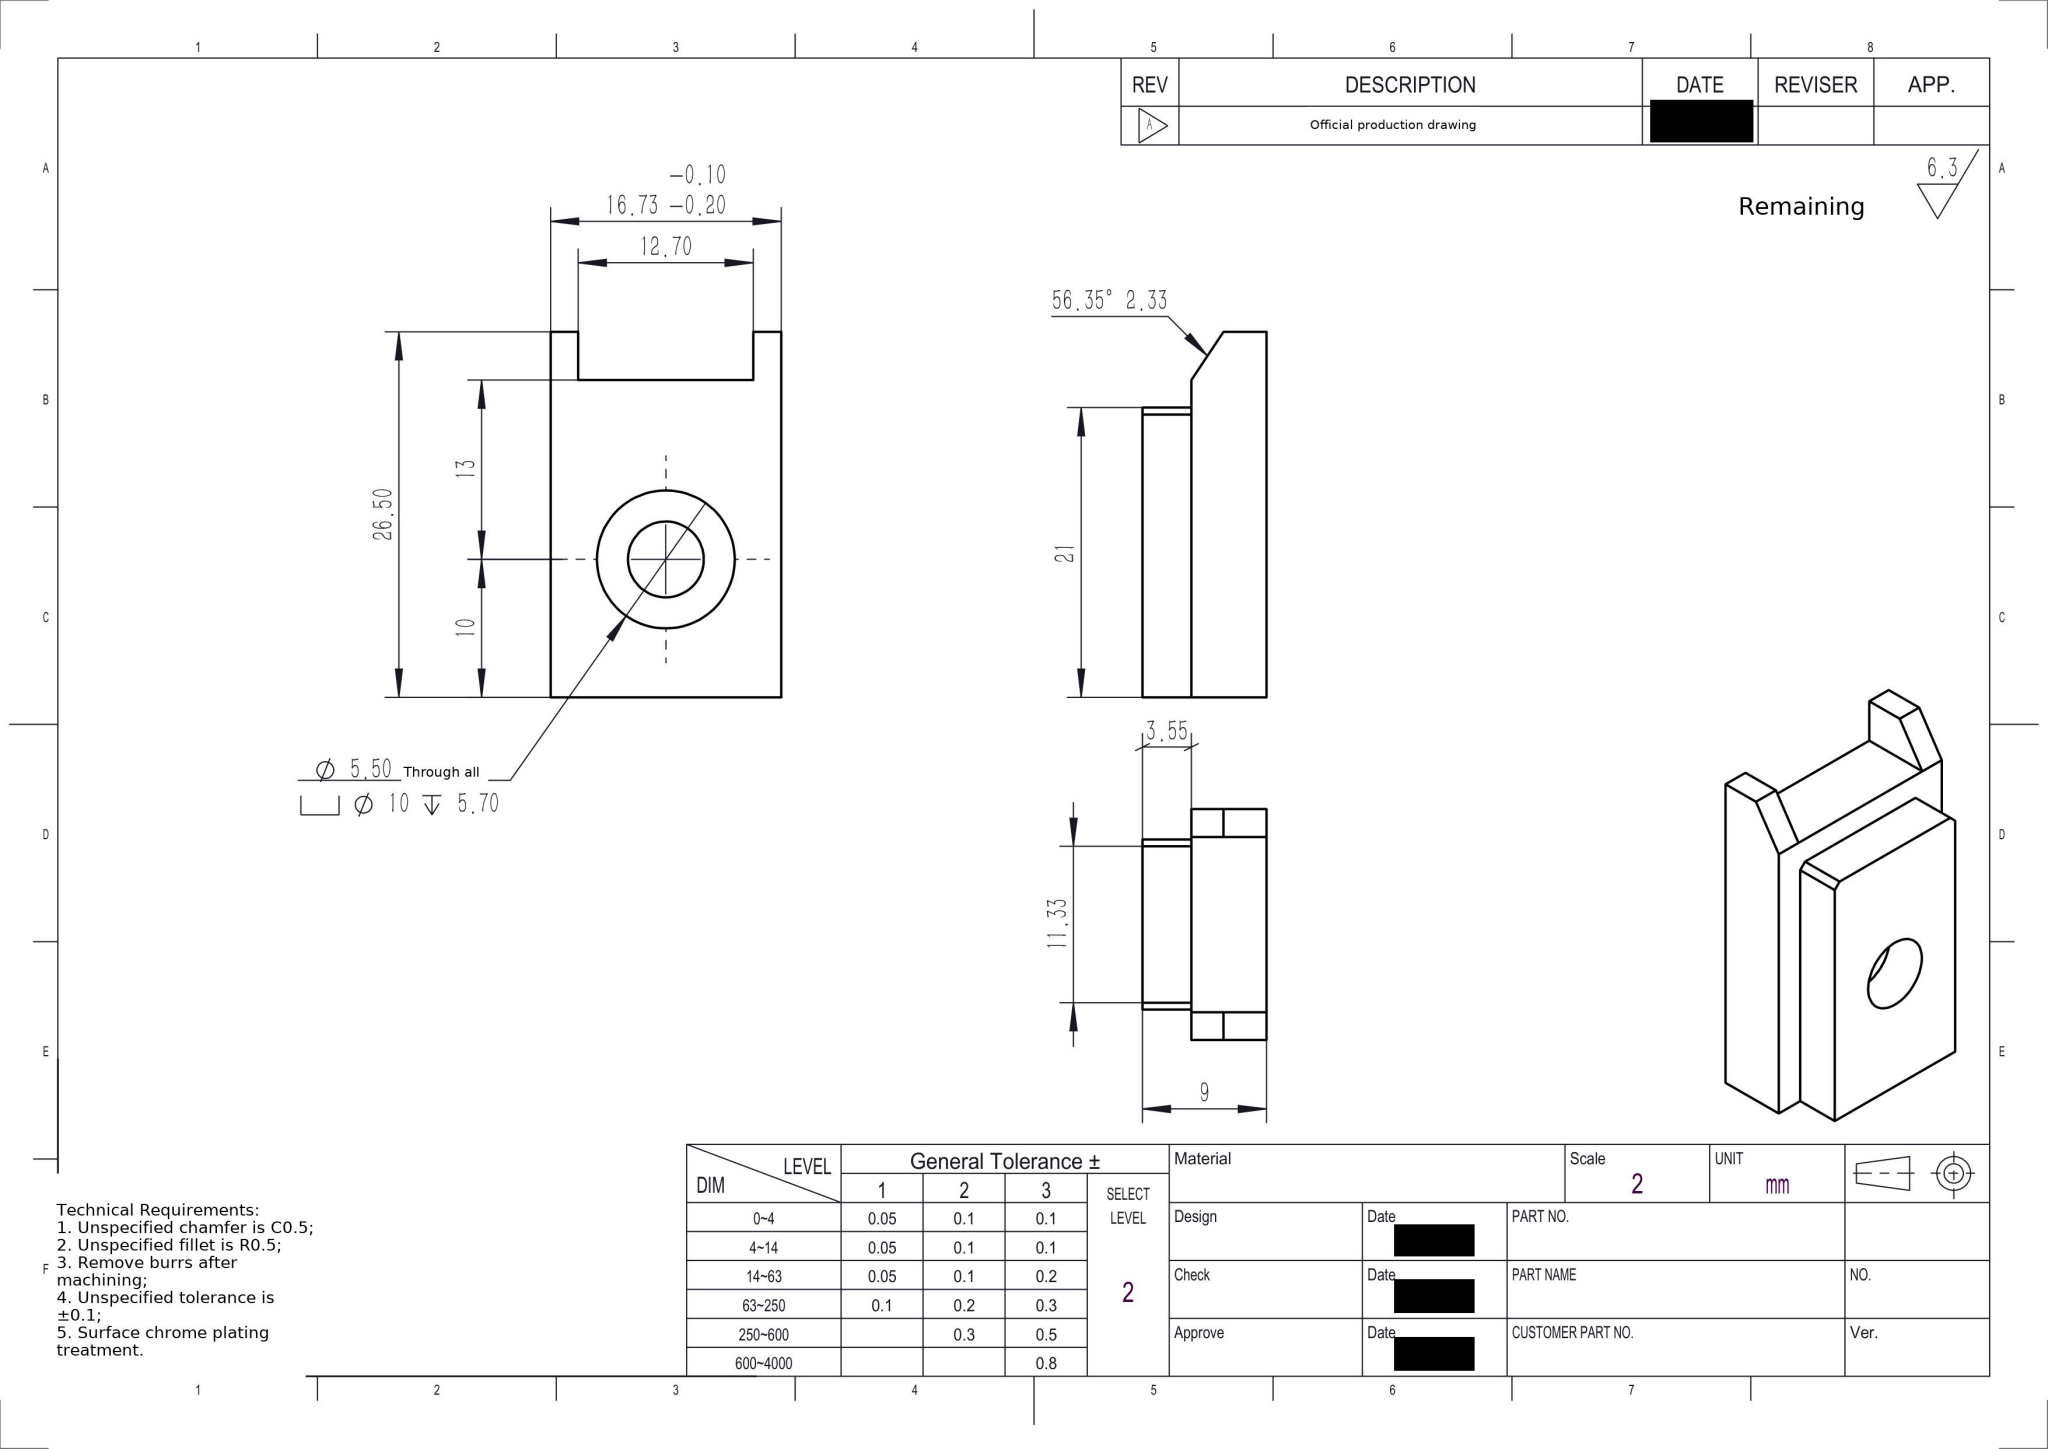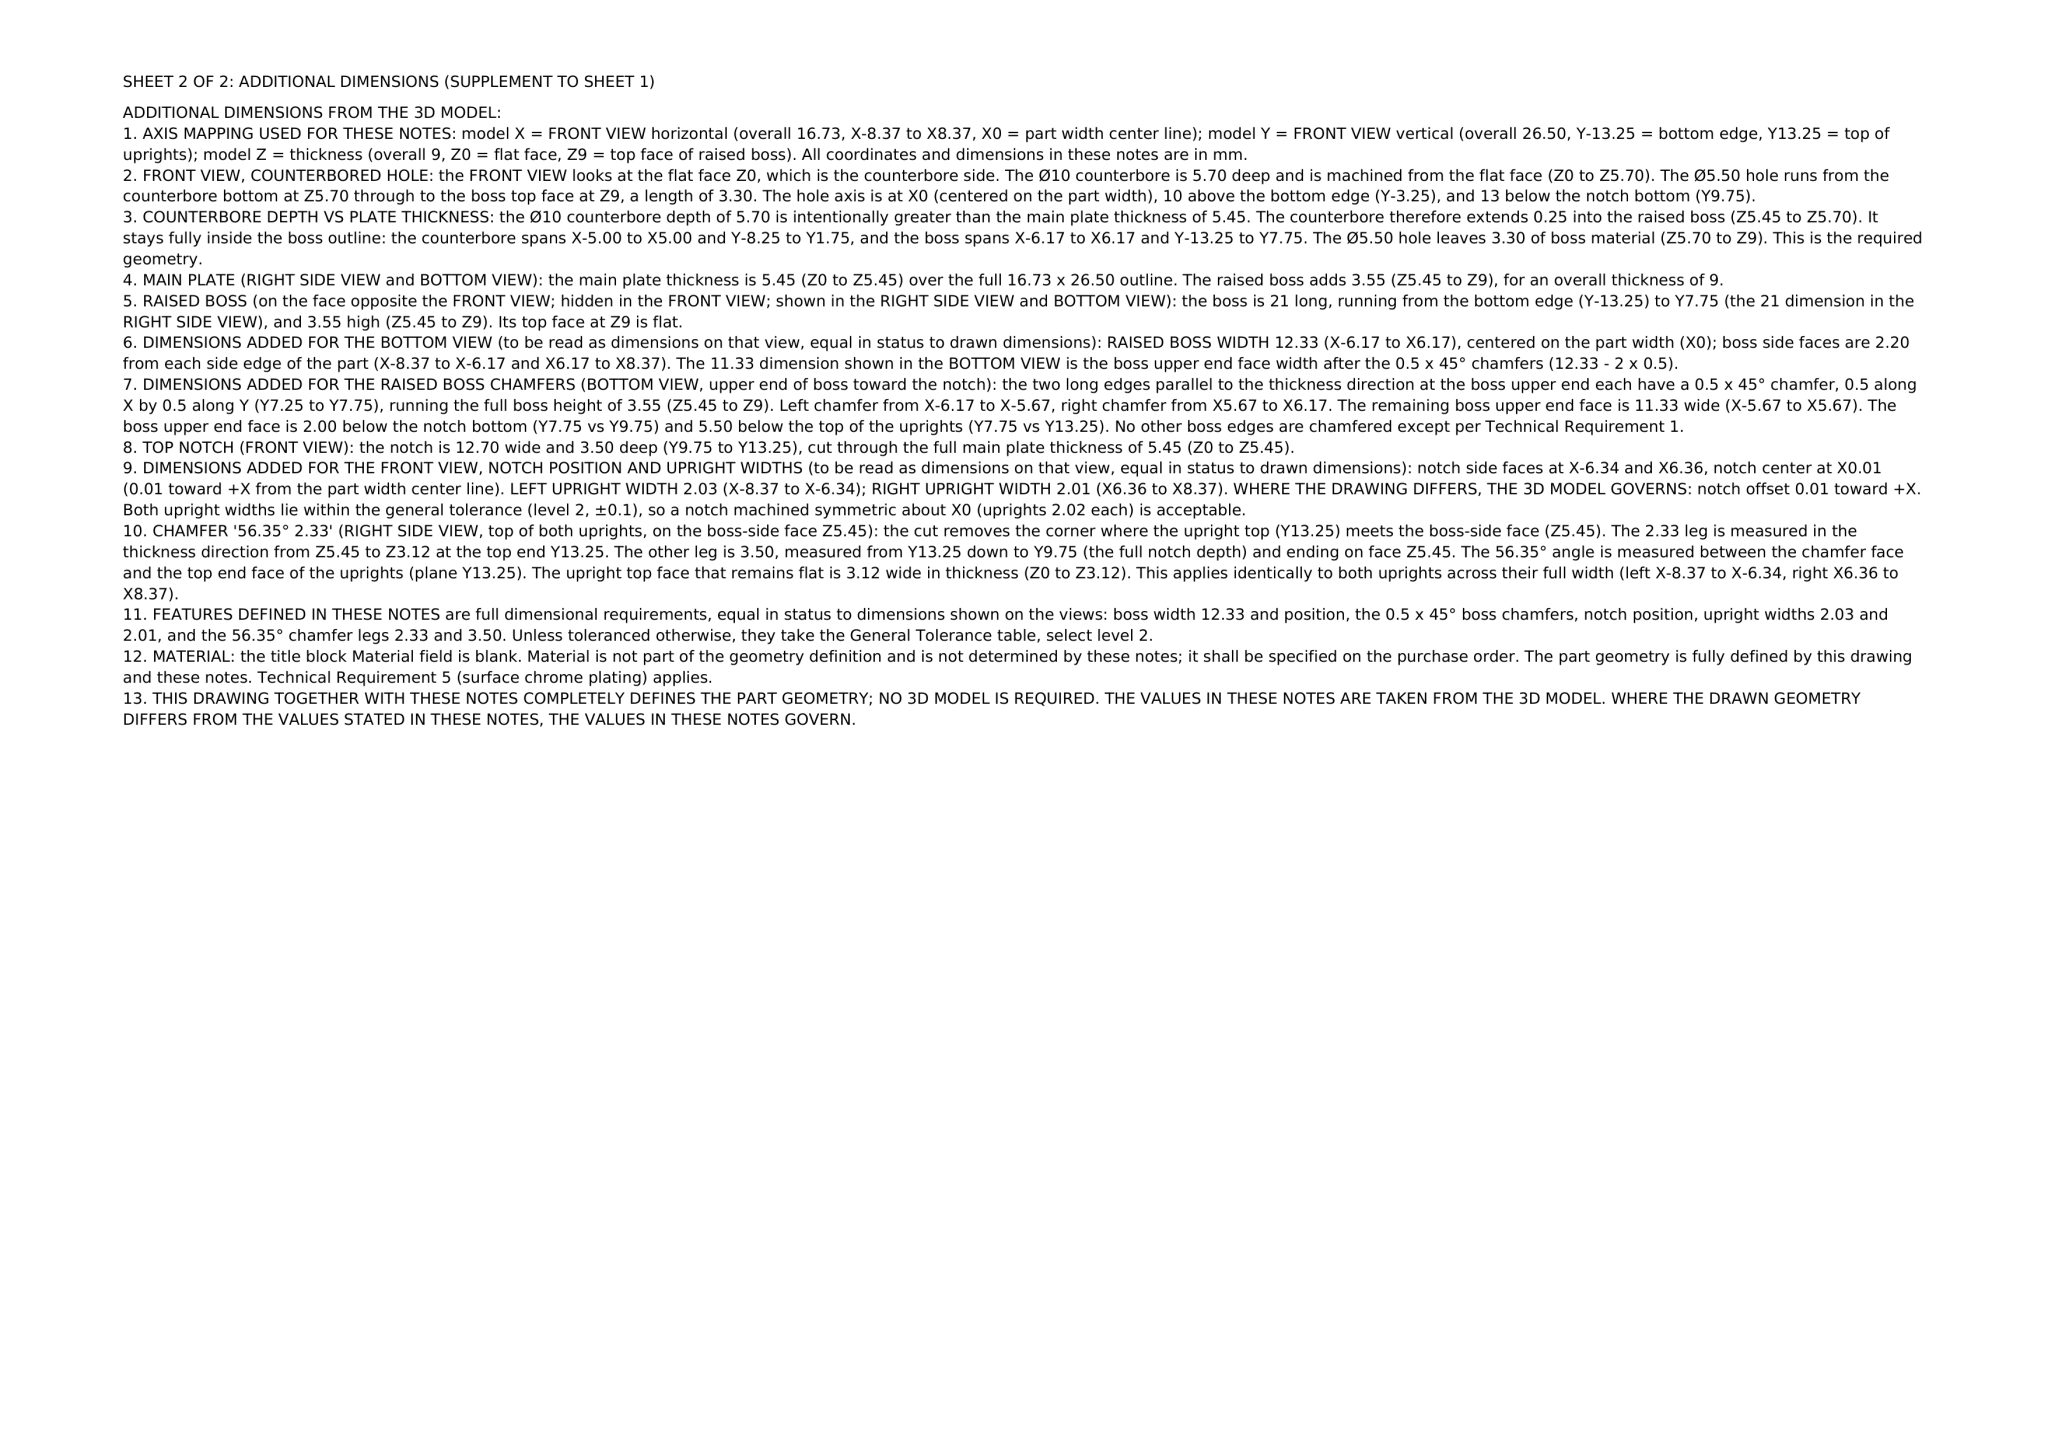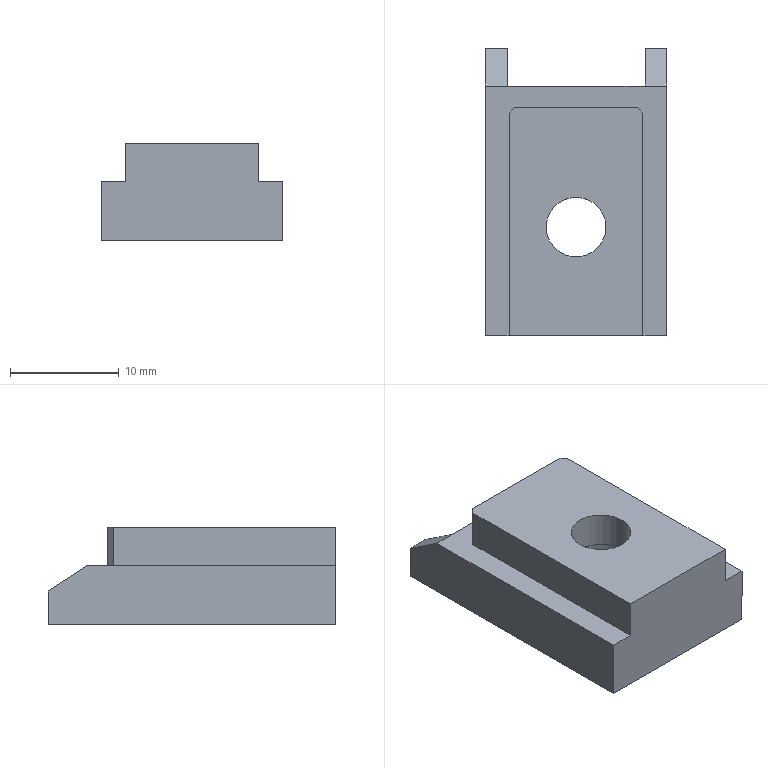Part | NX | mm | 396 | 1 solid | 23 faces | box 16.73 x 26.5 x 9 mm | volume 2550 mm3 | plane 19 | cylinder 4 | commonest cylinder face diameters 10 x2 5.5 x2
STEP:
#1=COLOUR_RGB('',0.7765,0.7569,0.7373);
#2=FILL_AREA_STYLE_COLOUR('',#1);
#3=FILL_AREA_STYLE('',(#2));
#4=SURFACE_STYLE_FILL_AREA(#3);
#5=SURFACE_SIDE_STYLE('',(#4));
#6=SURFACE_STYLE_USAGE(.BOTH.,#5);
#7=PRESENTATION_STYLE_ASSIGNMENT((#6));
#8=CARTESIAN_POINT('',(5.005,-3.25,5.7));
#9=VERTEX_POINT('',#8);
#10=CARTESIAN_POINT('',(-4.995,-3.25,5.7));
#11=VERTEX_POINT('',#10);
#12=CARTESIAN_POINT('',(0.005,-3.25,5.7));
#13=DIRECTION('',(0.,0.,-1.));
#14=DIRECTION('',(-1.,0.,0.));
#15=AXIS2_PLACEMENT_3D('',#12,#13,#14);
#16=CIRCLE('',#15,5.);
#17=EDGE_CURVE('',#9,#11,#16,.T.);
#18=ORIENTED_EDGE('',*,*,#17,.F.);
#19=CARTESIAN_POINT('',(5.005,-3.25,-0.));
#20=VERTEX_POINT('',#19);
#21=CARTESIAN_POINT('',(5.005,-3.25,0.));
#22=DIRECTION('',(0.,0.,-1.));
#23=VECTOR('',#22,1000.);
#24=LINE('',#21,#23);
#25=EDGE_CURVE('',#9,#20,#24,.T.);
#26=ORIENTED_EDGE('',*,*,#25,.T.);
#27=CARTESIAN_POINT('',(-4.995,-3.25,-0.));
#28=VERTEX_POINT('',#27);
#29=CARTESIAN_POINT('',(0.005,-3.25,-0.));
#30=DIRECTION('',(0.,0.,-1.));
#31=DIRECTION('',(-1.,0.,0.));
#32=AXIS2_PLACEMENT_3D('',#29,#30,#31);
#33=CIRCLE('',#32,5.);
#34=EDGE_CURVE('',#20,#28,#33,.T.);
#35=ORIENTED_EDGE('',*,*,#34,.T.);
#36=CARTESIAN_POINT('',(-4.995,-3.25,0.));
#37=DIRECTION('',(0.,0.,-1.));
#38=VECTOR('',#37,1000.);
#39=LINE('',#36,#38);
#40=EDGE_CURVE('',#11,#28,#39,.T.);
#41=ORIENTED_EDGE('',*,*,#40,.F.);
#42=EDGE_LOOP('',(#18,#26,#35,#41));
#43=FACE_OUTER_BOUND('',#42,.T.);
#44=CARTESIAN_POINT('',(0.005,-3.25,0.));
#45=DIRECTION('',(0.,0.,-1.));
#46=DIRECTION('',(-1.,0.,0.));
#47=AXIS2_PLACEMENT_3D('',#44,#45,#46);
#48=CYLINDRICAL_SURFACE('',#47,5.);
#49=ADVANCED_FACE('',(#43),#48,.F.);
#50=CARTESIAN_POINT('',(2.755,-3.25,9.));
#51=VERTEX_POINT('',#50);
#52=CARTESIAN_POINT('',(-2.745,-3.25,9.));
#53=VERTEX_POINT('',#52);
#54=CARTESIAN_POINT('',(0.005,-3.25,9.));
#55=DIRECTION('',(0.,0.,-1.));
#56=DIRECTION('',(-1.,0.,0.));
#57=AXIS2_PLACEMENT_3D('',#54,#55,#56);
#58=CIRCLE('',#57,2.75);
#59=EDGE_CURVE('',#51,#53,#58,.T.);
#60=ORIENTED_EDGE('',*,*,#59,.F.);
#61=CARTESIAN_POINT('',(2.755,-3.25,5.7));
#62=VERTEX_POINT('',#61);
#63=CARTESIAN_POINT('',(2.755,-3.25,0.));
#64=DIRECTION('',(0.,0.,-1.));
#65=VECTOR('',#64,1000.);
#66=LINE('',#63,#65);
#67=EDGE_CURVE('',#51,#62,#66,.T.);
#68=ORIENTED_EDGE('',*,*,#67,.T.);
#69=CARTESIAN_POINT('',(-2.745,-3.25,5.7));
#70=VERTEX_POINT('',#69);
#71=CARTESIAN_POINT('',(0.005,-3.25,5.7));
#72=DIRECTION('',(0.,0.,-1.));
#73=DIRECTION('',(-1.,0.,0.));
#74=AXIS2_PLACEMENT_3D('',#71,#72,#73);
#75=CIRCLE('',#74,2.75);
#76=EDGE_CURVE('',#62,#70,#75,.T.);
#77=ORIENTED_EDGE('',*,*,#76,.T.);
#78=CARTESIAN_POINT('',(-2.745,-3.25,0.));
#79=DIRECTION('',(0.,0.,-1.));
#80=VECTOR('',#79,1000.);
#81=LINE('',#78,#80);
#82=EDGE_CURVE('',#53,#70,#81,.T.);
#83=ORIENTED_EDGE('',*,*,#82,.F.);
#84=EDGE_LOOP('',(#60,#68,#77,#83));
#85=FACE_OUTER_BOUND('',#84,.T.);
#86=CARTESIAN_POINT('',(0.005,-3.25,0.));
#87=DIRECTION('',(0.,0.,-1.));
#88=DIRECTION('',(-1.,0.,0.));
#89=AXIS2_PLACEMENT_3D('',#86,#87,#88);
#90=CYLINDRICAL_SURFACE('',#89,2.75);
#91=ADVANCED_FACE('',(#85),#90,.F.);
#92=CARTESIAN_POINT('',(8.365,13.25,0.));
#93=VERTEX_POINT('',#92);
#94=CARTESIAN_POINT('',(6.365,13.25,0.));
#95=VERTEX_POINT('',#94);
#96=CARTESIAN_POINT('',(-8.365,13.25,0.));
#97=DIRECTION('',(-1.,0.,0.));
#98=VECTOR('',#97,1000.);
#99=LINE('',#96,#98);
#100=EDGE_CURVE('',#93,#95,#99,.T.);
#101=ORIENTED_EDGE('',*,*,#100,.T.);
#102=CARTESIAN_POINT('',(6.365,13.25,3.12));
#103=VERTEX_POINT('',#102);
#104=CARTESIAN_POINT('',(6.365,13.25,9.));
#105=DIRECTION('',(0.,0.,-1.));
#106=VECTOR('',#105,1000.);
#107=LINE('',#104,#106);
#108=EDGE_CURVE('',#103,#95,#107,.T.);
#109=ORIENTED_EDGE('',*,*,#108,.F.);
#110=CARTESIAN_POINT('',(8.365,13.25,3.12));
#111=VERTEX_POINT('',#110);
#112=CARTESIAN_POINT('',(-8.365,13.25,3.12));
#113=DIRECTION('',(1.,0.,0.));
#114=VECTOR('',#113,1000.);
#115=LINE('',#112,#114);
#116=EDGE_CURVE('',#103,#111,#115,.T.);
#117=ORIENTED_EDGE('',*,*,#116,.T.);
#118=CARTESIAN_POINT('',(8.365,13.25,9.));
#119=DIRECTION('',(0.,0.,-1.));
#120=VECTOR('',#119,1000.);
#121=LINE('',#118,#120);
#122=EDGE_CURVE('',#111,#93,#121,.T.);
#123=ORIENTED_EDGE('',*,*,#122,.T.);
#124=EDGE_LOOP('',(#101,#109,#117,#123));
#125=FACE_OUTER_BOUND('',#124,.T.);
#126=CARTESIAN_POINT('',(-8.365,13.25,9.));
#127=DIRECTION('',(0.,-1.,0.));
#128=DIRECTION('',(0.,0.,-1.));
#129=AXIS2_PLACEMENT_3D('',#126,#127,#128);
#130=PLANE('',#129);
#131=ADVANCED_FACE('',(#125),#130,.F.);
#132=ORIENTED_EDGE('',*,*,#116,.F.);
#133=CARTESIAN_POINT('',(6.365,9.75,5.45));
#134=VERTEX_POINT('',#133);
#135=CARTESIAN_POINT('',(6.365,13.25,3.12));
#136=DIRECTION('',(0.,-0.8324,0.5542));
#137=VECTOR('',#136,1000.);
#138=LINE('',#135,#137);
#139=EDGE_CURVE('',#103,#134,#138,.T.);
#140=ORIENTED_EDGE('',*,*,#139,.T.);
#141=CARTESIAN_POINT('',(8.365,9.75,5.45));
#142=VERTEX_POINT('',#141);
#143=CARTESIAN_POINT('',(-8.365,9.75,5.45));
#144=DIRECTION('',(1.,0.,0.));
#145=VECTOR('',#144,1000.);
#146=LINE('',#143,#145);
#147=EDGE_CURVE('',#134,#142,#146,.T.);
#148=ORIENTED_EDGE('',*,*,#147,.T.);
#149=CARTESIAN_POINT('',(8.365,13.25,3.12));
#150=DIRECTION('',(0.,0.8324,-0.5542));
#151=VECTOR('',#150,1000.);
#152=LINE('',#149,#151);
#153=EDGE_CURVE('',#142,#111,#152,.T.);
#154=ORIENTED_EDGE('',*,*,#153,.T.);
#155=EDGE_LOOP('',(#132,#140,#148,#154));
#156=FACE_OUTER_BOUND('',#155,.T.);
#157=CARTESIAN_POINT('',(-8.365,13.25,3.12));
#158=DIRECTION('',(0.,-0.5542,-0.8324));
#159=DIRECTION('',(0.,0.8324,-0.5542));
#160=AXIS2_PLACEMENT_3D('',#157,#158,#159);
#161=PLANE('',#160);
#162=ADVANCED_FACE('',(#156),#161,.F.);
#163=CARTESIAN_POINT('',(8.365,-13.25,5.45));
#164=VERTEX_POINT('',#163);
#165=CARTESIAN_POINT('',(8.365,9.75,5.45));
#166=DIRECTION('',(0.,1.,0.));
#167=VECTOR('',#166,1000.);
#168=LINE('',#165,#167);
#169=EDGE_CURVE('',#164,#142,#168,.T.);
#170=ORIENTED_EDGE('',*,*,#169,.F.);
#171=CARTESIAN_POINT('',(8.365,-13.25,0.));
#172=VERTEX_POINT('',#171);
#173=CARTESIAN_POINT('',(8.365,-13.25,9.));
#174=DIRECTION('',(0.,0.,-1.));
#175=VECTOR('',#174,1000.);
#176=LINE('',#173,#175);
#177=EDGE_CURVE('',#164,#172,#176,.T.);
#178=ORIENTED_EDGE('',*,*,#177,.T.);
#179=CARTESIAN_POINT('',(8.365,13.25,0.));
#180=DIRECTION('',(0.,1.,0.));
#181=VECTOR('',#180,1000.);
#182=LINE('',#179,#181);
#183=EDGE_CURVE('',#172,#93,#182,.T.);
#184=ORIENTED_EDGE('',*,*,#183,.T.);
#185=ORIENTED_EDGE('',*,*,#122,.F.);
#186=ORIENTED_EDGE('',*,*,#153,.F.);
#187=EDGE_LOOP('',(#170,#178,#184,#185,#186));
#188=FACE_OUTER_BOUND('',#187,.T.);
#189=CARTESIAN_POINT('',(8.365,13.25,9.));
#190=DIRECTION('',(-1.,0.,0.));
#191=DIRECTION('',(0.,0.,1.));
#192=AXIS2_PLACEMENT_3D('',#189,#190,#191);
#193=PLANE('',#192);
#194=ADVANCED_FACE('',(#188),#193,.F.);
#195=CARTESIAN_POINT('',(-8.365,13.25,3.12));
#196=VERTEX_POINT('',#195);
#197=CARTESIAN_POINT('',(-6.335,13.25,3.12));
#198=VERTEX_POINT('',#197);
#199=CARTESIAN_POINT('',(-8.365,13.25,3.12));
#200=DIRECTION('',(1.,0.,0.));
#201=VECTOR('',#200,1000.);
#202=LINE('',#199,#201);
#203=EDGE_CURVE('',#196,#198,#202,.T.);
#204=ORIENTED_EDGE('',*,*,#203,.T.);
#205=CARTESIAN_POINT('',(-6.335,13.25,0.));
#206=VERTEX_POINT('',#205);
#207=CARTESIAN_POINT('',(-6.335,13.25,9.));
#208=DIRECTION('',(0.,0.,-1.));
#209=VECTOR('',#208,1000.);
#210=LINE('',#207,#209);
#211=EDGE_CURVE('',#198,#206,#210,.T.);
#212=ORIENTED_EDGE('',*,*,#211,.T.);
#213=CARTESIAN_POINT('',(-8.365,13.25,0.));
#214=VERTEX_POINT('',#213);
#215=CARTESIAN_POINT('',(-8.365,13.25,0.));
#216=DIRECTION('',(-1.,0.,0.));
#217=VECTOR('',#216,1000.);
#218=LINE('',#215,#217);
#219=EDGE_CURVE('',#206,#214,#218,.T.);
#220=ORIENTED_EDGE('',*,*,#219,.T.);
#221=CARTESIAN_POINT('',(-8.365,13.25,9.));
#222=DIRECTION('',(0.,0.,-1.));
#223=VECTOR('',#222,1000.);
#224=LINE('',#221,#223);
#225=EDGE_CURVE('',#196,#214,#224,.T.);
#226=ORIENTED_EDGE('',*,*,#225,.F.);
#227=EDGE_LOOP('',(#204,#212,#220,#226));
#228=FACE_OUTER_BOUND('',#227,.T.);
#229=CARTESIAN_POINT('',(-8.365,13.25,9.));
#230=DIRECTION('',(0.,-1.,0.));
#231=DIRECTION('',(0.,0.,-1.));
#232=AXIS2_PLACEMENT_3D('',#229,#230,#231);
#233=PLANE('',#232);
#234=ADVANCED_FACE('',(#228),#233,.F.);
#235=CARTESIAN_POINT('',(-8.365,-13.25,5.45));
#236=VERTEX_POINT('',#235);
#237=CARTESIAN_POINT('',(-8.365,-13.25,0.));
#238=VERTEX_POINT('',#237);
#239=CARTESIAN_POINT('',(-8.365,-13.25,9.));
#240=DIRECTION('',(0.,0.,-1.));
#241=VECTOR('',#240,1000.);
#242=LINE('',#239,#241);
#243=EDGE_CURVE('',#236,#238,#242,.T.);
#244=ORIENTED_EDGE('',*,*,#243,.F.);
#245=CARTESIAN_POINT('',(-8.365,9.75,5.45));
#246=VERTEX_POINT('',#245);
#247=CARTESIAN_POINT('',(-8.365,9.75,5.45));
#248=DIRECTION('',(0.,1.,0.));
#249=VECTOR('',#248,1000.);
#250=LINE('',#247,#249);
#251=EDGE_CURVE('',#236,#246,#250,.T.);
#252=ORIENTED_EDGE('',*,*,#251,.T.);
#253=CARTESIAN_POINT('',(-8.365,13.25,3.12));
#254=DIRECTION('',(0.,0.8324,-0.5542));
#255=VECTOR('',#254,1000.);
#256=LINE('',#253,#255);
#257=EDGE_CURVE('',#246,#196,#256,.T.);
#258=ORIENTED_EDGE('',*,*,#257,.T.);
#259=ORIENTED_EDGE('',*,*,#225,.T.);
#260=CARTESIAN_POINT('',(-8.365,13.25,0.));
#261=DIRECTION('',(0.,-1.,0.));
#262=VECTOR('',#261,1000.);
#263=LINE('',#260,#262);
#264=EDGE_CURVE('',#214,#238,#263,.T.);
#265=ORIENTED_EDGE('',*,*,#264,.T.);
#266=EDGE_LOOP('',(#244,#252,#258,#259,#265));
#267=FACE_OUTER_BOUND('',#266,.T.);
#268=CARTESIAN_POINT('',(-8.365,13.25,9.));
#269=DIRECTION('',(1.,0.,0.));
#270=DIRECTION('',(-0.,1.,0.));
#271=AXIS2_PLACEMENT_3D('',#268,#269,#270);
#272=PLANE('',#271);
#273=ADVANCED_FACE('',(#267),#272,.F.);
#274=CARTESIAN_POINT('',(-6.165,-13.25,9.));
#275=VERTEX_POINT('',#274);
#276=CARTESIAN_POINT('',(-6.165,-13.25,5.45));
#277=VERTEX_POINT('',#276);
#278=CARTESIAN_POINT('',(-6.165,-13.25,9.));
#279=DIRECTION('',(0.,0.,-1.));
#280=VECTOR('',#279,1000.);
#281=LINE('',#278,#280);
#282=EDGE_CURVE('',#275,#277,#281,.T.);
#283=ORIENTED_EDGE('',*,*,#282,.T.);
#284=CARTESIAN_POINT('',(-8.365,-13.25,5.45));
#285=DIRECTION('',(-1.,0.,0.));
#286=VECTOR('',#285,1000.);
#287=LINE('',#284,#286);
#288=EDGE_CURVE('',#277,#236,#287,.T.);
#289=ORIENTED_EDGE('',*,*,#288,.T.);
#290=ORIENTED_EDGE('',*,*,#243,.T.);
#291=CARTESIAN_POINT('',(-8.365,-13.25,0.));
#292=DIRECTION('',(1.,0.,0.));
#293=VECTOR('',#292,1000.);
#294=LINE('',#291,#293);
#295=EDGE_CURVE('',#238,#172,#294,.T.);
#296=ORIENTED_EDGE('',*,*,#295,.T.);
#297=ORIENTED_EDGE('',*,*,#177,.F.);
#298=CARTESIAN_POINT('',(6.165,-13.25,5.45));
#299=VERTEX_POINT('',#298);
#300=CARTESIAN_POINT('',(8.365,-13.25,5.45));
#301=DIRECTION('',(-1.,0.,-0.));
#302=VECTOR('',#301,1000.);
#303=LINE('',#300,#302);
#304=EDGE_CURVE('',#164,#299,#303,.T.);
#305=ORIENTED_EDGE('',*,*,#304,.T.);
#306=CARTESIAN_POINT('',(6.165,-13.25,9.));
#307=VERTEX_POINT('',#306);
#308=CARTESIAN_POINT('',(6.165,-13.25,9.));
#309=DIRECTION('',(0.,0.,1.));
#310=VECTOR('',#309,1000.);
#311=LINE('',#308,#310);
#312=EDGE_CURVE('',#299,#307,#311,.T.);
#313=ORIENTED_EDGE('',*,*,#312,.T.);
#314=CARTESIAN_POINT('',(-8.365,-13.25,9.));
#315=DIRECTION('',(1.,0.,0.));
#316=VECTOR('',#315,1000.);
#317=LINE('',#314,#316);
#318=EDGE_CURVE('',#275,#307,#317,.T.);
#319=ORIENTED_EDGE('',*,*,#318,.F.);
#320=EDGE_LOOP('',(#283,#289,#290,#296,#297,#305,#313,#319));
#321=FACE_OUTER_BOUND('',#320,.T.);
#322=CARTESIAN_POINT('',(-8.365,-13.25,9.));
#323=DIRECTION('',(0.,1.,0.));
#324=DIRECTION('',(0.,0.,1.));
#325=AXIS2_PLACEMENT_3D('',#322,#323,#324);
#326=PLANE('',#325);
#327=ADVANCED_FACE('',(#321),#326,.F.);
#328=CARTESIAN_POINT('',(6.165,7.25,9.));
#329=VERTEX_POINT('',#328);
#330=CARTESIAN_POINT('',(6.165,-13.25,9.));
#331=DIRECTION('',(0.,1.,0.));
#332=VECTOR('',#331,1000.);
#333=LINE('',#330,#332);
#334=EDGE_CURVE('',#307,#329,#333,.T.);
#335=ORIENTED_EDGE('',*,*,#334,.T.);
#336=CARTESIAN_POINT('',(5.665,7.75,9.));
#337=VERTEX_POINT('',#336);
#338=CARTESIAN_POINT('',(6.708,6.708,9.));
#339=DIRECTION('',(-0.7071,0.7071,0.));
#340=VECTOR('',#339,1000.);
#341=LINE('',#338,#340);
#342=EDGE_CURVE('',#329,#337,#341,.T.);
#343=ORIENTED_EDGE('',*,*,#342,.T.);
#344=CARTESIAN_POINT('',(-5.665,7.75,9.));
#345=VERTEX_POINT('',#344);
#346=CARTESIAN_POINT('',(-8.365,7.75,9.));
#347=DIRECTION('',(1.,0.,0.));
#348=VECTOR('',#347,1000.);
#349=LINE('',#346,#348);
#350=EDGE_CURVE('',#345,#337,#349,.T.);
#351=ORIENTED_EDGE('',*,*,#350,.F.);
#352=CARTESIAN_POINT('',(-6.165,7.25,9.));
#353=VERTEX_POINT('',#352);
#354=CARTESIAN_POINT('',(-6.708,6.708,9.));
#355=DIRECTION('',(-0.7071,-0.7071,0.));
#356=VECTOR('',#355,1000.);
#357=LINE('',#354,#356);
#358=EDGE_CURVE('',#345,#353,#357,.T.);
#359=ORIENTED_EDGE('',*,*,#358,.T.);
#360=CARTESIAN_POINT('',(-6.165,-13.25,9.));
#361=DIRECTION('',(0.,1.,0.));
#362=VECTOR('',#361,1000.);
#363=LINE('',#360,#362);
#364=EDGE_CURVE('',#275,#353,#363,.T.);
#365=ORIENTED_EDGE('',*,*,#364,.F.);
#366=ORIENTED_EDGE('',*,*,#318,.T.);
#367=EDGE_LOOP('',(#335,#343,#351,#359,#365,#366));
#368=FACE_OUTER_BOUND('',#367,.T.);
#369=CARTESIAN_POINT('',(0.005,-3.25,9.));
#370=DIRECTION('',(0.,0.,-1.));
#371=DIRECTION('',(-1.,0.,0.));
#372=AXIS2_PLACEMENT_3D('',#369,#370,#371);
#373=CIRCLE('',#372,2.75);
#374=EDGE_CURVE('',#53,#51,#373,.T.);
#375=ORIENTED_EDGE('',*,*,#374,.T.);
#376=ORIENTED_EDGE('',*,*,#59,.T.);
#377=EDGE_LOOP('',(#375,#376));
#378=FACE_BOUND('',#377,.T.);
#379=CARTESIAN_POINT('',(0.,0.,9.));
#380=DIRECTION('',(0.,0.,1.));
#381=DIRECTION('',(1.,0.,0.));
#382=AXIS2_PLACEMENT_3D('',#379,#380,#381);
#383=PLANE('',#382);
#384=ADVANCED_FACE('',(#368,#378),#383,.T.);
#385=CARTESIAN_POINT('',(0.005,-3.25,-0.));
#386=DIRECTION('',(0.,0.,-1.));
#387=DIRECTION('',(-1.,0.,0.));
#388=AXIS2_PLACEMENT_3D('',#385,#386,#387);
#389=CIRCLE('',#388,5.);
#390=EDGE_CURVE('',#28,#20,#389,.T.);
#391=ORIENTED_EDGE('',*,*,#390,.F.);
#392=ORIENTED_EDGE('',*,*,#34,.F.);
#393=EDGE_LOOP('',(#391,#392));
#394=FACE_BOUND('',#393,.T.);
#395=CARTESIAN_POINT('',(6.365,9.75,0.));
#396=VERTEX_POINT('',#395);
#397=CARTESIAN_POINT('',(-6.335,9.75,0.));
#398=VERTEX_POINT('',#397);
#399=CARTESIAN_POINT('',(6.365,9.75,0.));
#400=DIRECTION('',(-1.,-0.,0.));
#401=VECTOR('',#400,1000.);
#402=LINE('',#399,#401);
#403=EDGE_CURVE('',#396,#398,#402,.T.);
#404=ORIENTED_EDGE('',*,*,#403,.F.);
#405=CARTESIAN_POINT('',(6.365,13.25,0.));
#406=DIRECTION('',(0.,-1.,0.));
#407=VECTOR('',#406,1000.);
#408=LINE('',#405,#407);
#409=EDGE_CURVE('',#95,#396,#408,.T.);
#410=ORIENTED_EDGE('',*,*,#409,.F.);
#411=ORIENTED_EDGE('',*,*,#100,.F.);
#412=ORIENTED_EDGE('',*,*,#183,.F.);
#413=ORIENTED_EDGE('',*,*,#295,.F.);
#414=ORIENTED_EDGE('',*,*,#264,.F.);
#415=ORIENTED_EDGE('',*,*,#219,.F.);
#416=CARTESIAN_POINT('',(-6.335,13.25,0.));
#417=DIRECTION('',(0.,1.,0.));
#418=VECTOR('',#417,1000.);
#419=LINE('',#416,#418);
#420=EDGE_CURVE('',#398,#206,#419,.T.);
#421=ORIENTED_EDGE('',*,*,#420,.F.);
#422=EDGE_LOOP('',(#404,#410,#411,#412,#413,#414,#415,#421));
#423=FACE_OUTER_BOUND('',#422,.T.);
#424=CARTESIAN_POINT('',(0.,0.,0.));
#425=DIRECTION('',(0.,0.,1.));
#426=DIRECTION('',(1.,0.,0.));
#427=AXIS2_PLACEMENT_3D('',#424,#425,#426);
#428=PLANE('',#427);
#429=ADVANCED_FACE('',(#394,#423),#428,.F.);
#430=CARTESIAN_POINT('',(-6.335,9.75,5.45));
#431=VERTEX_POINT('',#430);
#432=CARTESIAN_POINT('',(-8.365,9.75,5.45));
#433=DIRECTION('',(1.,0.,0.));
#434=VECTOR('',#433,1000.);
#435=LINE('',#432,#434);
#436=EDGE_CURVE('',#246,#431,#435,.T.);
#437=ORIENTED_EDGE('',*,*,#436,.T.);
#438=CARTESIAN_POINT('',(-6.335,13.25,3.12));
#439=DIRECTION('',(0.,0.8324,-0.5542));
#440=VECTOR('',#439,1000.);
#441=LINE('',#438,#440);
#442=EDGE_CURVE('',#431,#198,#441,.T.);
#443=ORIENTED_EDGE('',*,*,#442,.T.);
#444=ORIENTED_EDGE('',*,*,#203,.F.);
#445=ORIENTED_EDGE('',*,*,#257,.F.);
#446=EDGE_LOOP('',(#437,#443,#444,#445));
#447=FACE_OUTER_BOUND('',#446,.T.);
#448=CARTESIAN_POINT('',(-8.365,13.25,3.12));
#449=DIRECTION('',(0.,-0.5542,-0.8324));
#450=DIRECTION('',(0.,0.8324,-0.5542));
#451=AXIS2_PLACEMENT_3D('',#448,#449,#450);
#452=PLANE('',#451);
#453=ADVANCED_FACE('',(#447),#452,.F.);
#454=ORIENTED_EDGE('',*,*,#169,.T.);
#455=ORIENTED_EDGE('',*,*,#147,.F.);
#456=CARTESIAN_POINT('',(-8.365,9.75,5.45));
#457=DIRECTION('',(1.,0.,0.));
#458=VECTOR('',#457,1000.);
#459=LINE('',#456,#458);
#460=EDGE_CURVE('',#431,#134,#459,.T.);
#461=ORIENTED_EDGE('',*,*,#460,.F.);
#462=ORIENTED_EDGE('',*,*,#436,.F.);
#463=ORIENTED_EDGE('',*,*,#251,.F.);
#464=ORIENTED_EDGE('',*,*,#288,.F.);
#465=CARTESIAN_POINT('',(-6.165,7.25,5.45));
#466=VERTEX_POINT('',#465);
#467=CARTESIAN_POINT('',(-6.165,-13.25,5.45));
#468=DIRECTION('',(0.,1.,0.));
#469=VECTOR('',#468,1000.);
#470=LINE('',#467,#469);
#471=EDGE_CURVE('',#277,#466,#470,.T.);
#472=ORIENTED_EDGE('',*,*,#471,.T.);
#473=CARTESIAN_POINT('',(-5.665,7.75,5.45));
#474=VERTEX_POINT('',#473);
#475=CARTESIAN_POINT('',(-6.015,7.4,5.45));
#476=DIRECTION('',(0.7071,0.7071,0.));
#477=VECTOR('',#476,1000.);
#478=LINE('',#475,#477);
#479=EDGE_CURVE('',#466,#474,#478,.T.);
#480=ORIENTED_EDGE('',*,*,#479,.T.);
#481=CARTESIAN_POINT('',(5.665,7.75,5.45));
#482=VERTEX_POINT('',#481);
#483=CARTESIAN_POINT('',(-8.365,7.75,5.45));
#484=DIRECTION('',(1.,0.,0.));
#485=VECTOR('',#484,1000.);
#486=LINE('',#483,#485);
#487=EDGE_CURVE('',#474,#482,#486,.T.);
#488=ORIENTED_EDGE('',*,*,#487,.T.);
#489=CARTESIAN_POINT('',(6.165,7.25,5.45));
#490=VERTEX_POINT('',#489);
#491=CARTESIAN_POINT('',(-2.35,15.765,5.45));
#492=DIRECTION('',(0.7071,-0.7071,0.));
#493=VECTOR('',#492,1000.);
#494=LINE('',#491,#493);
#495=EDGE_CURVE('',#482,#490,#494,.T.);
#496=ORIENTED_EDGE('',*,*,#495,.T.);
#497=CARTESIAN_POINT('',(6.165,-13.25,5.45));
#498=DIRECTION('',(0.,1.,0.));
#499=VECTOR('',#498,1000.);
#500=LINE('',#497,#499);
#501=EDGE_CURVE('',#299,#490,#500,.T.);
#502=ORIENTED_EDGE('',*,*,#501,.F.);
#503=ORIENTED_EDGE('',*,*,#304,.F.);
#504=EDGE_LOOP('',(#454,#455,#461,#462,#463,#464,#472,#480,#488,#496,#502,#503));
#505=FACE_OUTER_BOUND('',#504,.T.);
#506=CARTESIAN_POINT('',(-8.365,9.75,5.45));
#507=DIRECTION('',(0.,0.,-1.));
#508=DIRECTION('',(-1.,0.,0.));
#509=AXIS2_PLACEMENT_3D('',#506,#507,#508);
#510=PLANE('',#509);
#511=ADVANCED_FACE('',(#505),#510,.F.);
#512=ORIENTED_EDGE('',*,*,#350,.T.);
#513=CARTESIAN_POINT('',(5.665,7.75,5.45));
#514=DIRECTION('',(0.,0.,-1.));
#515=VECTOR('',#514,1000.);
#516=LINE('',#513,#515);
#517=EDGE_CURVE('',#337,#482,#516,.T.);
#518=ORIENTED_EDGE('',*,*,#517,.T.);
#519=ORIENTED_EDGE('',*,*,#487,.F.);
#520=CARTESIAN_POINT('',(-5.665,7.75,5.45));
#521=DIRECTION('',(0.,0.,1.));
#522=VECTOR('',#521,1000.);
#523=LINE('',#520,#522);
#524=EDGE_CURVE('',#474,#345,#523,.T.);
#525=ORIENTED_EDGE('',*,*,#524,.T.);
#526=EDGE_LOOP('',(#512,#518,#519,#525));
#527=FACE_OUTER_BOUND('',#526,.T.);
#528=CARTESIAN_POINT('',(-8.365,7.75,5.45));
#529=DIRECTION('',(0.,-1.,0.));
#530=DIRECTION('',(0.,0.,-1.));
#531=AXIS2_PLACEMENT_3D('',#528,#529,#530);
#532=PLANE('',#531);
#533=ADVANCED_FACE('',(#527),#532,.F.);
#534=ORIENTED_EDGE('',*,*,#67,.F.);
#535=ORIENTED_EDGE('',*,*,#374,.F.);
#536=ORIENTED_EDGE('',*,*,#82,.T.);
#537=CARTESIAN_POINT('',(0.005,-3.25,5.7));
#538=DIRECTION('',(0.,0.,-1.));
#539=DIRECTION('',(-1.,0.,0.));
#540=AXIS2_PLACEMENT_3D('',#537,#538,#539);
#541=CIRCLE('',#540,2.75);
#542=EDGE_CURVE('',#70,#62,#541,.T.);
#543=ORIENTED_EDGE('',*,*,#542,.T.);
#544=EDGE_LOOP('',(#534,#535,#536,#543));
#545=FACE_OUTER_BOUND('',#544,.T.);
#546=CARTESIAN_POINT('',(0.005,-3.25,0.));
#547=DIRECTION('',(0.,0.,-1.));
#548=DIRECTION('',(-1.,0.,0.));
#549=AXIS2_PLACEMENT_3D('',#546,#547,#548);
#550=CYLINDRICAL_SURFACE('',#549,2.75);
#551=ADVANCED_FACE('',(#545),#550,.F.);
#552=ORIENTED_EDGE('',*,*,#542,.F.);
#553=ORIENTED_EDGE('',*,*,#76,.F.);
#554=EDGE_LOOP('',(#552,#553));
#555=FACE_BOUND('',#554,.T.);
#556=CARTESIAN_POINT('',(0.005,-3.25,5.7));
#557=DIRECTION('',(0.,0.,-1.));
#558=DIRECTION('',(-1.,0.,0.));
#559=AXIS2_PLACEMENT_3D('',#556,#557,#558);
#560=CIRCLE('',#559,5.);
#561=EDGE_CURVE('',#11,#9,#560,.T.);
#562=ORIENTED_EDGE('',*,*,#561,.T.);
#563=ORIENTED_EDGE('',*,*,#17,.T.);
#564=EDGE_LOOP('',(#562,#563));
#565=FACE_OUTER_BOUND('',#564,.T.);
#566=CARTESIAN_POINT('',(2.755,-3.25,5.7));
#567=DIRECTION('',(0.,0.,1.));
#568=DIRECTION('',(1.,0.,0.));
#569=AXIS2_PLACEMENT_3D('',#566,#567,#568);
#570=PLANE('',#569);
#571=ADVANCED_FACE('',(#555,#565),#570,.F.);
#572=ORIENTED_EDGE('',*,*,#25,.F.);
#573=ORIENTED_EDGE('',*,*,#561,.F.);
#574=ORIENTED_EDGE('',*,*,#40,.T.);
#575=ORIENTED_EDGE('',*,*,#390,.T.);
#576=EDGE_LOOP('',(#572,#573,#574,#575));
#577=FACE_OUTER_BOUND('',#576,.T.);
#578=CARTESIAN_POINT('',(0.005,-3.25,0.));
#579=DIRECTION('',(0.,0.,-1.));
#580=DIRECTION('',(-1.,0.,0.));
#581=AXIS2_PLACEMENT_3D('',#578,#579,#580);
#582=CYLINDRICAL_SURFACE('',#581,5.);
#583=ADVANCED_FACE('',(#577),#582,.F.);
#584=ORIENTED_EDGE('',*,*,#108,.T.);
#585=ORIENTED_EDGE('',*,*,#409,.T.);
#586=CARTESIAN_POINT('',(6.365,9.75,9.));
#587=DIRECTION('',(0.,0.,-1.));
#588=VECTOR('',#587,1000.);
#589=LINE('',#586,#588);
#590=EDGE_CURVE('',#134,#396,#589,.T.);
#591=ORIENTED_EDGE('',*,*,#590,.F.);
#592=ORIENTED_EDGE('',*,*,#139,.F.);
#593=EDGE_LOOP('',(#584,#585,#591,#592));
#594=FACE_OUTER_BOUND('',#593,.T.);
#595=CARTESIAN_POINT('',(6.365,13.25,9.));
#596=DIRECTION('',(1.,0.,0.));
#597=DIRECTION('',(0.,0.,-1.));
#598=AXIS2_PLACEMENT_3D('',#595,#596,#597);
#599=PLANE('',#598);
#600=ADVANCED_FACE('',(#594),#599,.F.);
#601=CARTESIAN_POINT('',(-6.335,9.75,9.));
#602=DIRECTION('',(0.,0.,-1.));
#603=VECTOR('',#602,1000.);
#604=LINE('',#601,#603);
#605=EDGE_CURVE('',#431,#398,#604,.T.);
#606=ORIENTED_EDGE('',*,*,#605,.T.);
#607=ORIENTED_EDGE('',*,*,#420,.T.);
#608=ORIENTED_EDGE('',*,*,#211,.F.);
#609=ORIENTED_EDGE('',*,*,#442,.F.);
#610=EDGE_LOOP('',(#606,#607,#608,#609));
#611=FACE_OUTER_BOUND('',#610,.T.);
#612=CARTESIAN_POINT('',(-6.335,13.25,9.));
#613=DIRECTION('',(-1.,0.,0.));
#614=DIRECTION('',(-0.,-1.,0.));
#615=AXIS2_PLACEMENT_3D('',#612,#613,#614);
#616=PLANE('',#615);
#617=ADVANCED_FACE('',(#611),#616,.F.);
#618=ORIENTED_EDGE('',*,*,#590,.T.);
#619=ORIENTED_EDGE('',*,*,#403,.T.);
#620=ORIENTED_EDGE('',*,*,#605,.F.);
#621=ORIENTED_EDGE('',*,*,#460,.T.);
#622=EDGE_LOOP('',(#618,#619,#620,#621));
#623=FACE_OUTER_BOUND('',#622,.T.);
#624=CARTESIAN_POINT('',(6.365,9.75,9.));
#625=DIRECTION('',(0.,-1.,0.));
#626=DIRECTION('',(1.,0.,0.));
#627=AXIS2_PLACEMENT_3D('',#624,#625,#626);
#628=PLANE('',#627);
#629=ADVANCED_FACE('',(#623),#628,.F.);
#630=ORIENTED_EDGE('',*,*,#501,.T.);
#631=CARTESIAN_POINT('',(6.165,7.25,9.));
#632=DIRECTION('',(0.,0.,1.));
#633=VECTOR('',#632,1000.);
#634=LINE('',#631,#633);
#635=EDGE_CURVE('',#490,#329,#634,.T.);
#636=ORIENTED_EDGE('',*,*,#635,.T.);
#637=ORIENTED_EDGE('',*,*,#334,.F.);
#638=ORIENTED_EDGE('',*,*,#312,.F.);
#639=EDGE_LOOP('',(#630,#636,#637,#638));
#640=FACE_OUTER_BOUND('',#639,.T.);
#641=CARTESIAN_POINT('',(6.165,-13.25,9.));
#642=DIRECTION('',(-1.,0.,0.));
#643=DIRECTION('',(0.,0.,1.));
#644=AXIS2_PLACEMENT_3D('',#641,#642,#643);
#645=PLANE('',#644);
#646=ADVANCED_FACE('',(#640),#645,.F.);
#647=ORIENTED_EDGE('',*,*,#364,.T.);
#648=CARTESIAN_POINT('',(-6.165,7.25,9.));
#649=DIRECTION('',(0.,0.,-1.));
#650=VECTOR('',#649,1000.);
#651=LINE('',#648,#650);
#652=EDGE_CURVE('',#353,#466,#651,.T.);
#653=ORIENTED_EDGE('',*,*,#652,.T.);
#654=ORIENTED_EDGE('',*,*,#471,.F.);
#655=ORIENTED_EDGE('',*,*,#282,.F.);
#656=EDGE_LOOP('',(#647,#653,#654,#655));
#657=FACE_OUTER_BOUND('',#656,.T.);
#658=CARTESIAN_POINT('',(-6.165,-13.25,9.));
#659=DIRECTION('',(1.,0.,0.));
#660=DIRECTION('',(0.,0.,-1.));
#661=AXIS2_PLACEMENT_3D('',#658,#659,#660);
#662=PLANE('',#661);
#663=ADVANCED_FACE('',(#657),#662,.F.);
#664=ORIENTED_EDGE('',*,*,#495,.F.);
#665=ORIENTED_EDGE('',*,*,#517,.F.);
#666=ORIENTED_EDGE('',*,*,#342,.F.);
#667=ORIENTED_EDGE('',*,*,#635,.F.);
#668=EDGE_LOOP('',(#664,#665,#666,#667));
#669=FACE_OUTER_BOUND('',#668,.T.);
#670=CARTESIAN_POINT('',(6.165,7.25,9.));
#671=DIRECTION('',(-0.7071,-0.7071,0.));
#672=DIRECTION('',(0.,0.,1.));
#673=AXIS2_PLACEMENT_3D('',#670,#671,#672);
#674=PLANE('',#673);
#675=ADVANCED_FACE('',(#669),#674,.F.);
#676=ORIENTED_EDGE('',*,*,#358,.F.);
#677=ORIENTED_EDGE('',*,*,#524,.F.);
#678=ORIENTED_EDGE('',*,*,#479,.F.);
#679=ORIENTED_EDGE('',*,*,#652,.F.);
#680=EDGE_LOOP('',(#676,#677,#678,#679));
#681=FACE_OUTER_BOUND('',#680,.T.);
#682=CARTESIAN_POINT('',(-6.165,7.25,9.));
#683=DIRECTION('',(0.7071,-0.7071,0.));
#684=DIRECTION('',(0.,0.,-1.));
#685=AXIS2_PLACEMENT_3D('',#682,#683,#684);
#686=PLANE('',#685);
#687=ADVANCED_FACE('',(#681),#686,.F.);
#688=CLOSED_SHELL('',(#49,#91,#131,#162,#194,#234,#273,#327,#384,#429,#453,#511,#533,#551,#571,#583,#600,#617,#629,#646,#663,#675,#687));
#689=MANIFOLD_SOLID_BREP('',#688);
#690=CARTESIAN_POINT('',(0.,0.,0.));
#691=DIRECTION('',(0.,0.,1.));
#692=DIRECTION('',(1.,0.,0.));
#693=AXIS2_PLACEMENT_3D('',#690,#691,#692);
#694=(LENGTH_UNIT()NAMED_UNIT(*)SI_UNIT(.MILLI.,.METRE.));
#695=UNCERTAINTY_MEASURE_WITH_UNIT(LENGTH_MEASURE(0.00001),#694,'','');
#696=(NAMED_UNIT(*)PLANE_ANGLE_UNIT()SI_UNIT($,.RADIAN.));
#697=(NAMED_UNIT(*)SI_UNIT($,.STERADIAN.)SOLID_ANGLE_UNIT());
#698=(GEOMETRIC_REPRESENTATION_CONTEXT(3)GLOBAL_UNCERTAINTY_ASSIGNED_CONTEXT((#695))GLOBAL_UNIT_ASSIGNED_CONTEXT((#694,#696,#697))REPRESENTATION_CONTEXT('',''));
#699=ADVANCED_BREP_SHAPE_REPRESENTATION('',(#689,#693),#698);
#700=STYLED_ITEM('',(#7),#699);
#701=(LENGTH_UNIT()NAMED_UNIT(*)SI_UNIT(.MILLI.,.METRE.));
#702=UNCERTAINTY_MEASURE_WITH_UNIT(LENGTH_MEASURE(0.00001),#701,'','');
#703=(NAMED_UNIT(*)PLANE_ANGLE_UNIT()SI_UNIT($,.RADIAN.));
#704=(NAMED_UNIT(*)SI_UNIT($,.STERADIAN.)SOLID_ANGLE_UNIT());
#705=(GEOMETRIC_REPRESENTATION_CONTEXT(3)GLOBAL_UNCERTAINTY_ASSIGNED_CONTEXT((#702))GLOBAL_UNIT_ASSIGNED_CONTEXT((#701,#703,#704))REPRESENTATION_CONTEXT('',''));
#706=MECHANICAL_DESIGN_GEOMETRIC_PRESENTATION_REPRESENTATION('',(#700),#705);
#707=COLOUR_RGB('',0.7765,0.7569,0.7373);
#708=FILL_AREA_STYLE_COLOUR('',#707);
#709=FILL_AREA_STYLE('',(#708));
#710=SURFACE_STYLE_FILL_AREA(#709);
#711=SURFACE_SIDE_STYLE('',(#710));
#712=SURFACE_STYLE_USAGE(.BOTH.,#711);
#713=PRESENTATION_STYLE_ASSIGNMENT((#712));
#714=STYLED_ITEM('',(#713),#689);
#715=(LENGTH_UNIT()NAMED_UNIT(*)SI_UNIT(.MILLI.,.METRE.));
#716=UNCERTAINTY_MEASURE_WITH_UNIT(LENGTH_MEASURE(0.00001),#715,'','');
#717=(NAMED_UNIT(*)PLANE_ANGLE_UNIT()SI_UNIT($,.RADIAN.));
#718=(NAMED_UNIT(*)SI_UNIT($,.STERADIAN.)SOLID_ANGLE_UNIT());
#719=(GEOMETRIC_REPRESENTATION_CONTEXT(3)GLOBAL_UNCERTAINTY_ASSIGNED_CONTEXT((#716))GLOBAL_UNIT_ASSIGNED_CONTEXT((#715,#717,#718))REPRESENTATION_CONTEXT('',''));
#720=MECHANICAL_DESIGN_GEOMETRIC_PRESENTATION_REPRESENTATION('',(#714),#719);
#721=PRESENTATION_LAYER_ASSIGNMENT('','',(#714));
#722=PRESENTATION_LAYER_ASSIGNMENT('','',(#700));